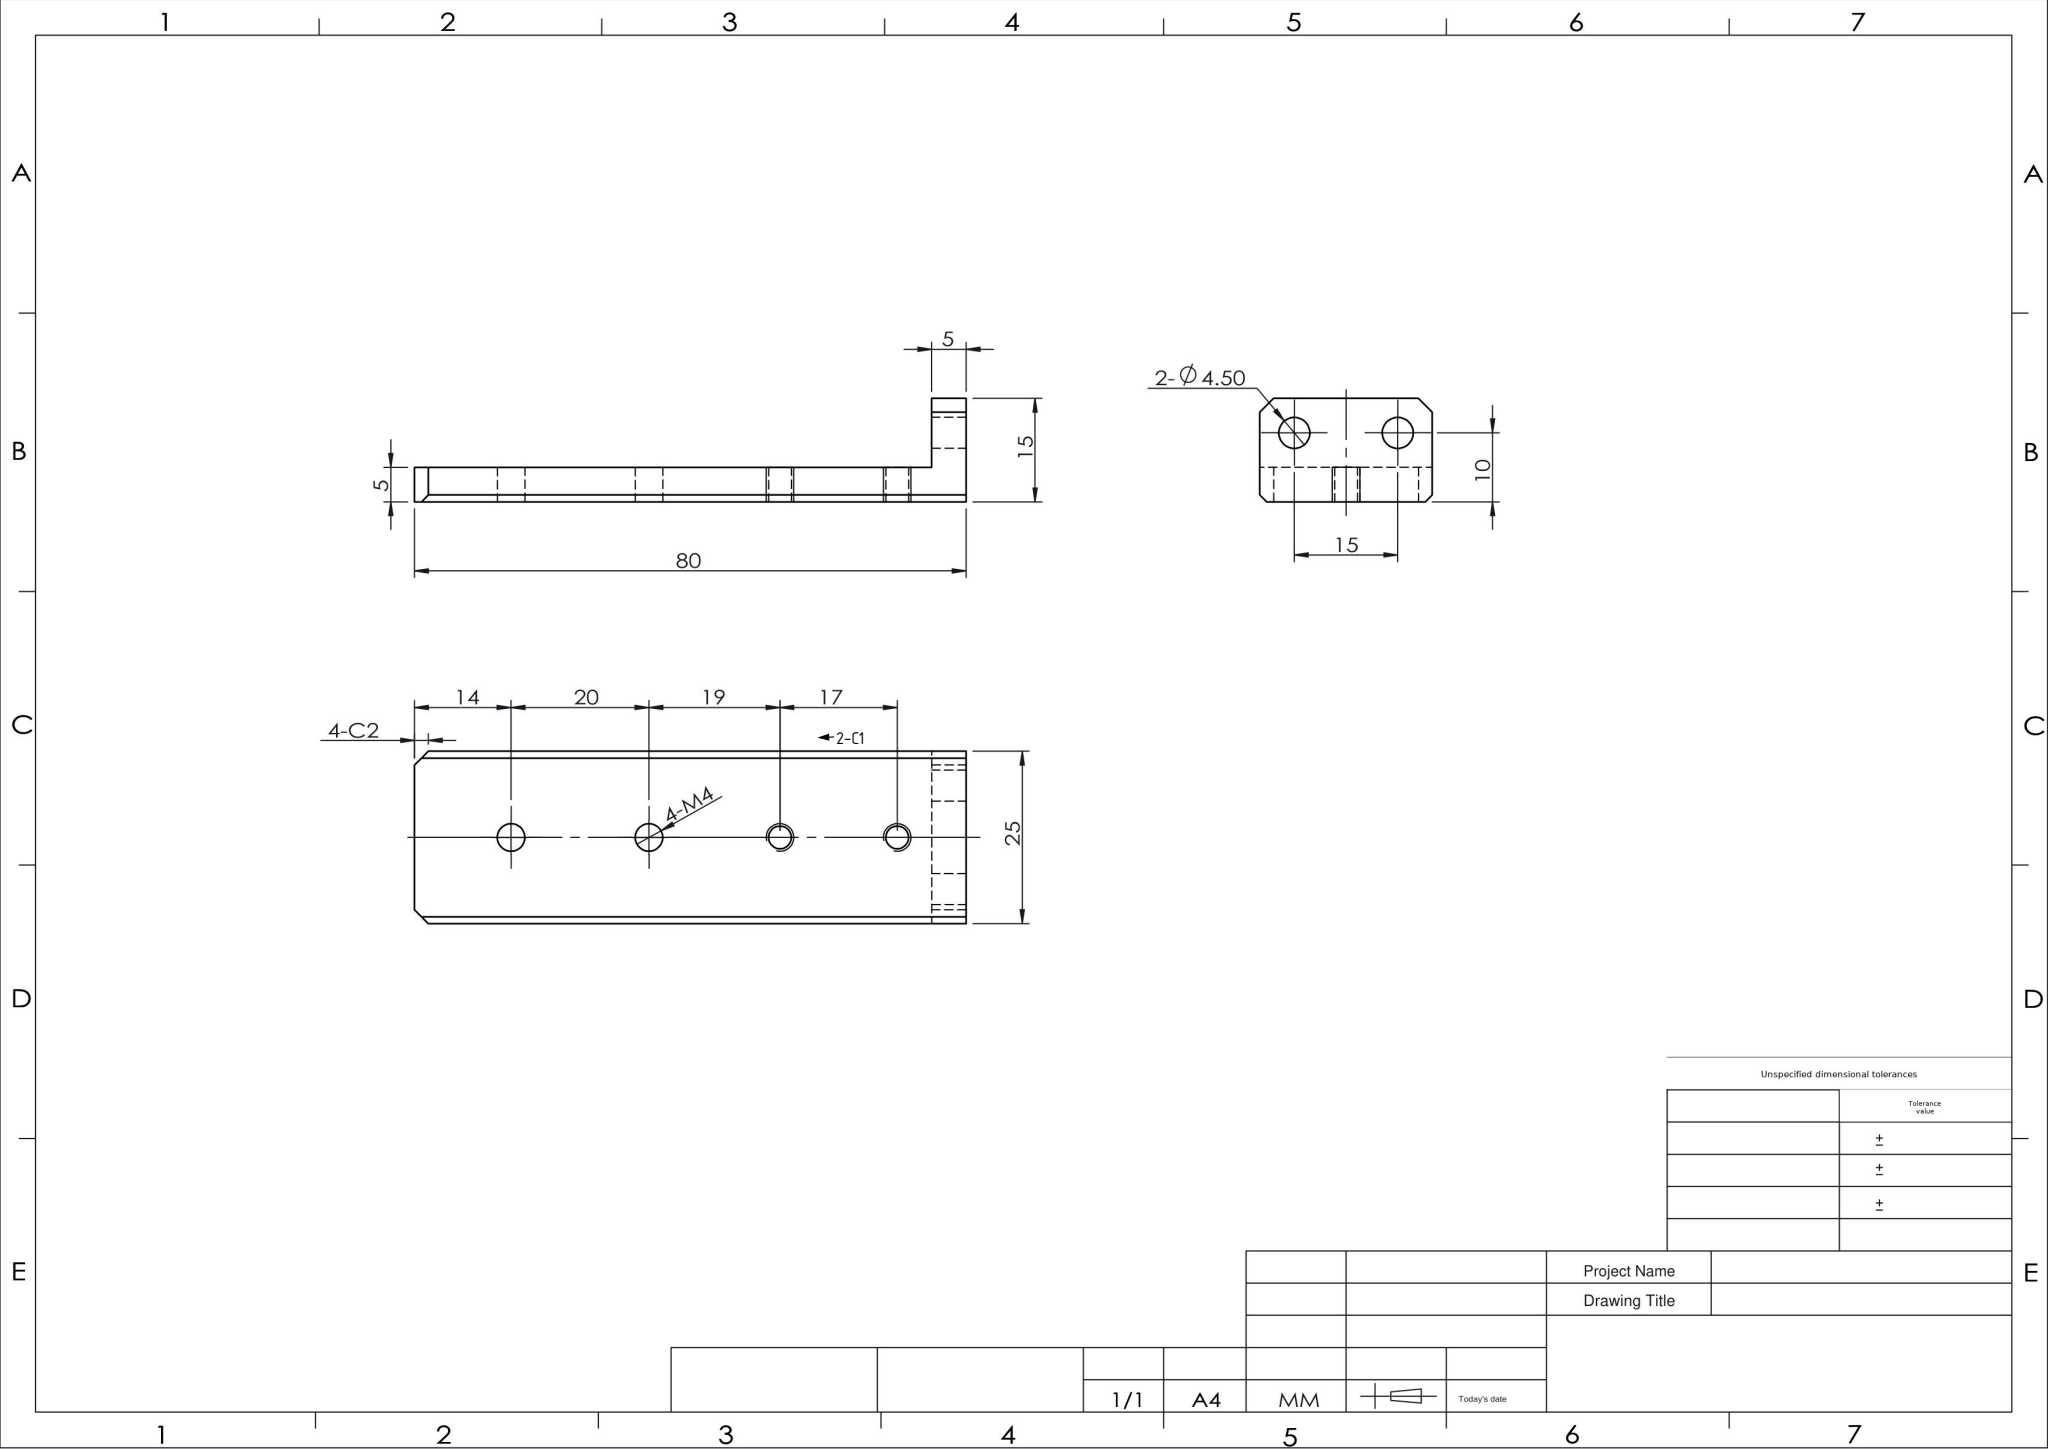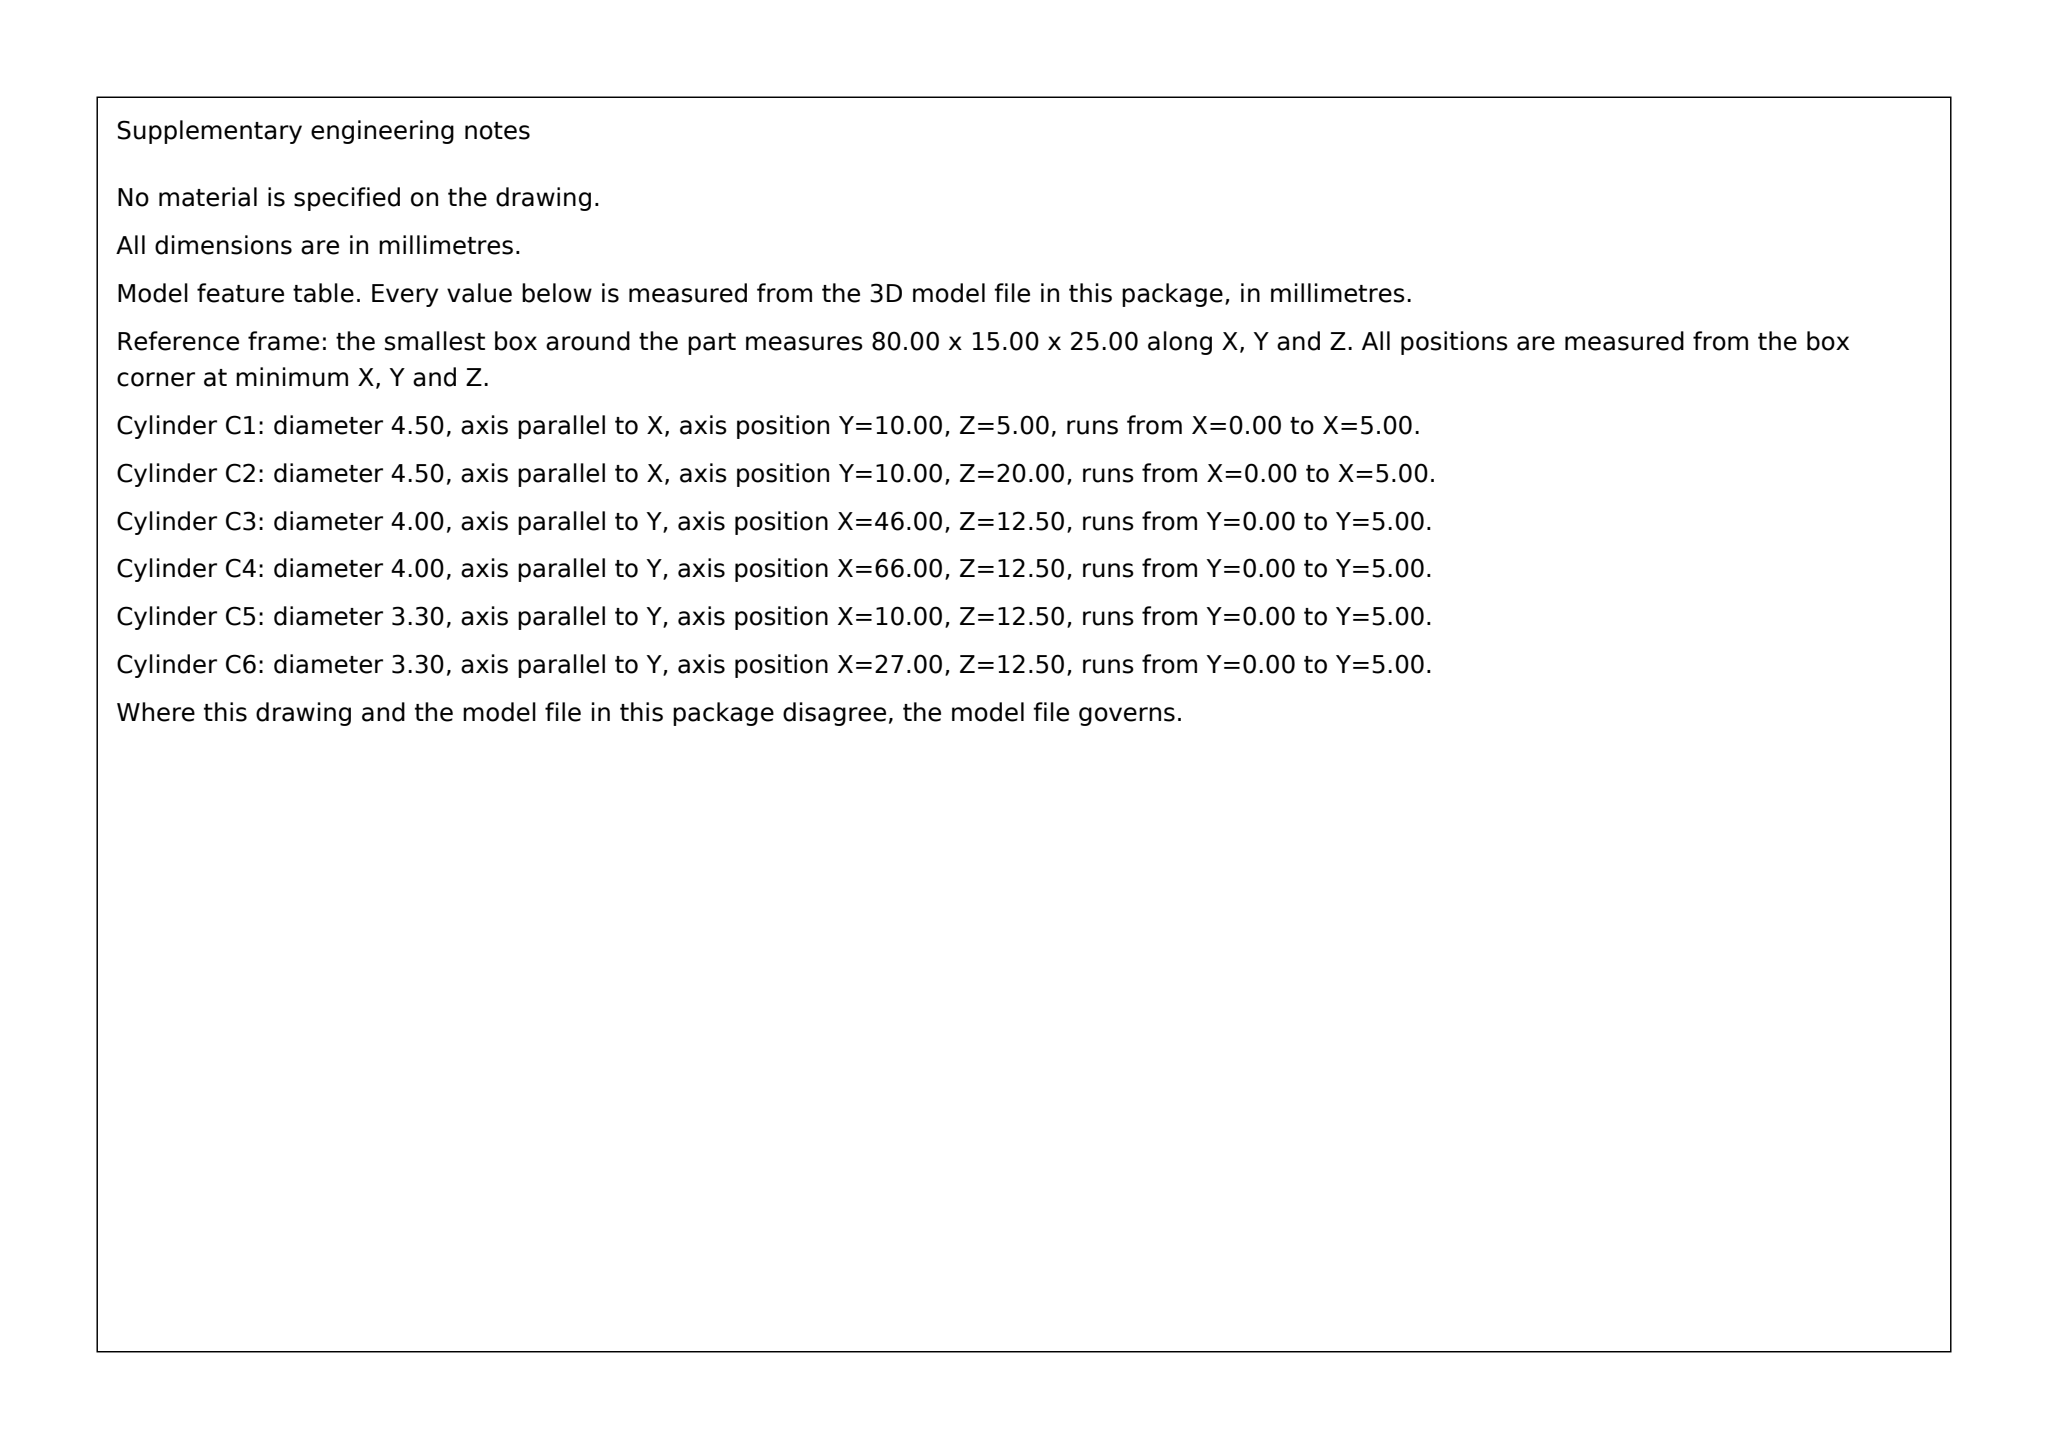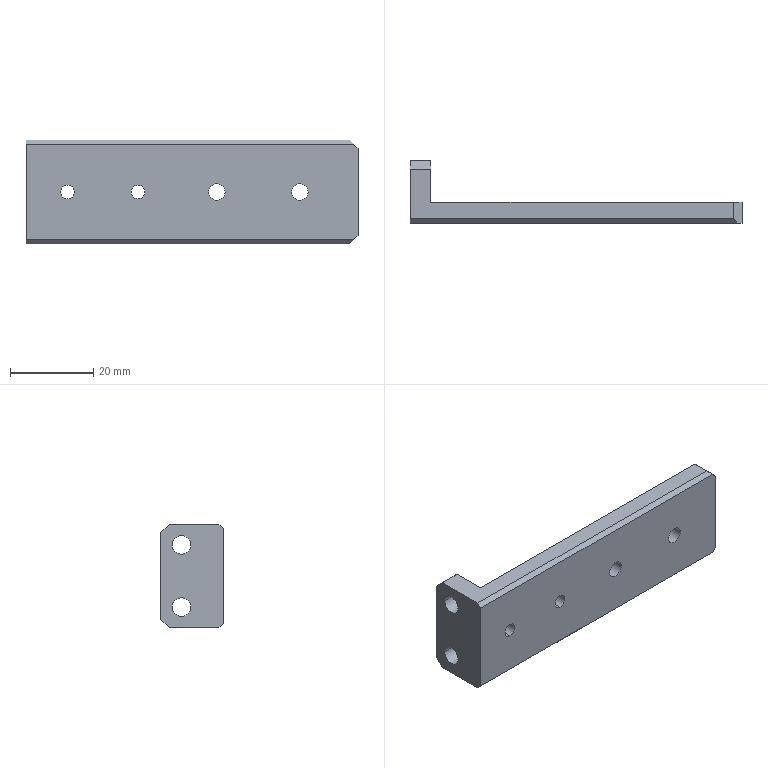Part | SolidWorks | mm | 1 solid | 26 faces | box 80 x 15 x 25 mm | volume 10761 mm3 | plane 14 | cylinder 12 | commonest cylinder face diameters 3.3 x4 4 x4 4.5 x4
Drawing notes:
2-C1 ON LONG BOTTOM EDGES OF 80 ARM (FRONT FACE, FULL 79 LG) | from the solid: Inclined planes 45/45 at bbox_from [0,0,0] and [0,0,24], size [79,1,1] -> 1x1 chamfers along x on y=0 face at z=0 and z=25
build123d program:
from build123d import *

# Parameters (mm, degrees)
BOSS_EXTRUDE1_DEPTH   = 25
SKETCH2_R             = 2.25
CUT_EXTRUDE1_DEPTH    = 81.467
CHAMFER1_SIZE         = 2
SKETCH3_R             = 2
CUT_EXTRUDE2_DEPTH    = 10
M4_TAPPED_HOLE1_D     = 3.3
M4_TAPPED_HOLE1_DEPTH = 10.1
M4_TAPPED_HOLE1_TIP   = 0.9914
CHAMFER2_SIZE         = 1


with BuildPart() as part:
    # Sketch1 → Boss-Extrude1 (new body)
    with BuildSketch(Plane.XY):
        Polygon((0, 15), (5, 15), (5, 5), (80, 5), (80, 0), (0, 0), align=None)
    extrude(amount=BOSS_EXTRUDE1_DEPTH)

    # Sketch2 → Cut-Extrude1 (cut, through all)
    with BuildSketch(Plane(origin=(5, 0, 0), x_dir=(0, 0, -1), z_dir=(1, 0, 0))):
        with Locations(Location((-20, 10, 0), (0, 0, 90))):
            Circle(SKETCH2_R)
        with Locations(Location((-5, 10, 0), (0, 0, 90))):
            Circle(SKETCH2_R)
    extrude(amount=-CUT_EXTRUDE1_DEPTH, mode=Mode.SUBTRACT)

    # Chamfer1
    chamfer1_edges = [part.edges().sort_by_distance(p)[0] for p in [
        (80, 2.5, 25),
        (2.5, 15, 25),
        (2.5, 15, 0),
        (80, 2.5, 0),
    ]]
    chamfer(chamfer1_edges, length=CHAMFER1_SIZE)

    # Sketch3 → Cut-Extrude2 (cut)
    with BuildSketch(Plane(origin=(0, 5, 0), x_dir=(1, 0, 0), z_dir=(0, 1, 0))):
        with Locations(Location((46, -12.5, 0), (0, 0, 180))):
            Circle(SKETCH3_R)
        with Locations(Location((66, -12.5, 0), (0, 0, 180))):
            Circle(SKETCH3_R)
    extrude(amount=-CUT_EXTRUDE2_DEPTH, mode=Mode.SUBTRACT)

    # M4 Tapped Hole1
    with Locations(Plane(origin=(0, 0, 0), x_dir=(-1, 0, 0), z_dir=(0, -1, 0))):
        with Locations((-10, -12.5), (-27, -12.5)):
            Hole(M4_TAPPED_HOLE1_D / 2, depth=M4_TAPPED_HOLE1_DEPTH)
            with Locations((0, 0, -(M4_TAPPED_HOLE1_DEPTH + M4_TAPPED_HOLE1_TIP / 2))):  # 118° drill point
                Cone(0, M4_TAPPED_HOLE1_D / 2, M4_TAPPED_HOLE1_TIP, mode=Mode.SUBTRACT)

    # Chamfer2
    chamfer2_edges = [part.edges().sort_by_distance(p)[0] for p in [
        (39, 0, 25),
        (39, 0, 0),
    ]]
    chamfer(chamfer2_edges, length=CHAMFER2_SIZE)


solid = part.part
STEP:
#1=CARTESIAN_POINT('',(10.,5.,14.15));
#2=VERTEX_POINT('',#1);
#3=CARTESIAN_POINT('',(10.,5.,10.85));
#4=VERTEX_POINT('',#3);
#5=CARTESIAN_POINT('',(10.,5.,12.5));
#6=DIRECTION('',(0.,-1.,0.));
#7=DIRECTION('',(0.,0.,-1.));
#8=AXIS2_PLACEMENT_3D('',#5,#6,#7);
#9=CIRCLE('',#8,1.65);
#10=EDGE_CURVE('',#2,#4,#9,.T.);
#11=ORIENTED_EDGE('',*,*,#10,.F.);
#12=CARTESIAN_POINT('',(10.,-0.,14.15));
#13=VERTEX_POINT('',#12);
#14=CARTESIAN_POINT('',(10.,0.,14.15));
#15=DIRECTION('',(0.,-1.,0.));
#16=VECTOR('',#15,1000.);
#17=LINE('',#14,#16);
#18=EDGE_CURVE('',#2,#13,#17,.T.);
#19=ORIENTED_EDGE('',*,*,#18,.T.);
#20=CARTESIAN_POINT('',(10.,-0.,10.85));
#21=VERTEX_POINT('',#20);
#22=CARTESIAN_POINT('',(10.,-0.,12.5));
#23=DIRECTION('',(0.,-1.,0.));
#24=DIRECTION('',(0.,0.,-1.));
#25=AXIS2_PLACEMENT_3D('',#22,#23,#24);
#26=CIRCLE('',#25,1.65);
#27=EDGE_CURVE('',#13,#21,#26,.T.);
#28=ORIENTED_EDGE('',*,*,#27,.T.);
#29=CARTESIAN_POINT('',(10.,0.,10.85));
#30=DIRECTION('',(0.,-1.,0.));
#31=VECTOR('',#30,1000.);
#32=LINE('',#29,#31);
#33=EDGE_CURVE('',#4,#21,#32,.T.);
#34=ORIENTED_EDGE('',*,*,#33,.F.);
#35=EDGE_LOOP('',(#11,#19,#28,#34));
#36=FACE_OUTER_BOUND('',#35,.T.);
#37=CARTESIAN_POINT('',(10.,0.,12.5));
#38=DIRECTION('',(0.,-1.,0.));
#39=DIRECTION('',(0.,0.,-1.));
#40=AXIS2_PLACEMENT_3D('',#37,#38,#39);
#41=CYLINDRICAL_SURFACE('',#40,1.65);
#42=ADVANCED_FACE('',(#36),#41,.F.);
#43=CARTESIAN_POINT('',(27.,5.,14.15));
#44=VERTEX_POINT('',#43);
#45=CARTESIAN_POINT('',(27.,5.,10.85));
#46=VERTEX_POINT('',#45);
#47=CARTESIAN_POINT('',(27.,5.,12.5));
#48=DIRECTION('',(0.,-1.,0.));
#49=DIRECTION('',(0.,0.,-1.));
#50=AXIS2_PLACEMENT_3D('',#47,#48,#49);
#51=CIRCLE('',#50,1.65);
#52=EDGE_CURVE('',#44,#46,#51,.T.);
#53=ORIENTED_EDGE('',*,*,#52,.F.);
#54=CARTESIAN_POINT('',(27.,-0.,14.15));
#55=VERTEX_POINT('',#54);
#56=CARTESIAN_POINT('',(27.,0.,14.15));
#57=DIRECTION('',(0.,-1.,0.));
#58=VECTOR('',#57,1000.);
#59=LINE('',#56,#58);
#60=EDGE_CURVE('',#44,#55,#59,.T.);
#61=ORIENTED_EDGE('',*,*,#60,.T.);
#62=CARTESIAN_POINT('',(27.,-0.,10.85));
#63=VERTEX_POINT('',#62);
#64=CARTESIAN_POINT('',(27.,-0.,12.5));
#65=DIRECTION('',(0.,-1.,0.));
#66=DIRECTION('',(0.,0.,-1.));
#67=AXIS2_PLACEMENT_3D('',#64,#65,#66);
#68=CIRCLE('',#67,1.65);
#69=EDGE_CURVE('',#55,#63,#68,.T.);
#70=ORIENTED_EDGE('',*,*,#69,.T.);
#71=CARTESIAN_POINT('',(27.,0.,10.85));
#72=DIRECTION('',(0.,-1.,0.));
#73=VECTOR('',#72,1000.);
#74=LINE('',#71,#73);
#75=EDGE_CURVE('',#46,#63,#74,.T.);
#76=ORIENTED_EDGE('',*,*,#75,.F.);
#77=EDGE_LOOP('',(#53,#61,#70,#76));
#78=FACE_OUTER_BOUND('',#77,.T.);
#79=CARTESIAN_POINT('',(27.,0.,12.5));
#80=DIRECTION('',(0.,-1.,0.));
#81=DIRECTION('',(0.,0.,-1.));
#82=AXIS2_PLACEMENT_3D('',#79,#80,#81);
#83=CYLINDRICAL_SURFACE('',#82,1.65);
#84=ADVANCED_FACE('',(#78),#83,.F.);
#85=CARTESIAN_POINT('',(68.,0.,12.5));
#86=VERTEX_POINT('',#85);
#87=CARTESIAN_POINT('',(64.,0.,12.5));
#88=VERTEX_POINT('',#87);
#89=CARTESIAN_POINT('',(66.,0.,12.5));
#90=DIRECTION('',(0.,1.,0.));
#91=DIRECTION('',(0.,0.,1.));
#92=AXIS2_PLACEMENT_3D('',#89,#90,#91);
#93=CIRCLE('',#92,2.);
#94=EDGE_CURVE('',#86,#88,#93,.T.);
#95=ORIENTED_EDGE('',*,*,#94,.F.);
#96=CARTESIAN_POINT('',(68.,5.,12.5));
#97=VERTEX_POINT('',#96);
#98=CARTESIAN_POINT('',(68.,-5.,12.5));
#99=DIRECTION('',(-0.,1.,0.));
#100=VECTOR('',#99,1000.);
#101=LINE('',#98,#100);
#102=EDGE_CURVE('',#86,#97,#101,.T.);
#103=ORIENTED_EDGE('',*,*,#102,.T.);
#104=CARTESIAN_POINT('',(64.,5.,12.5));
#105=VERTEX_POINT('',#104);
#106=CARTESIAN_POINT('',(66.,5.,12.5));
#107=DIRECTION('',(-0.,1.,0.));
#108=DIRECTION('',(-1.,0.,0.));
#109=AXIS2_PLACEMENT_3D('',#106,#107,#108);
#110=CIRCLE('',#109,2.);
#111=EDGE_CURVE('',#97,#105,#110,.T.);
#112=ORIENTED_EDGE('',*,*,#111,.T.);
#113=CARTESIAN_POINT('',(64.,-5.,12.5));
#114=DIRECTION('',(-0.,1.,0.));
#115=VECTOR('',#114,1000.);
#116=LINE('',#113,#115);
#117=EDGE_CURVE('',#88,#105,#116,.T.);
#118=ORIENTED_EDGE('',*,*,#117,.F.);
#119=EDGE_LOOP('',(#95,#103,#112,#118));
#120=FACE_OUTER_BOUND('',#119,.T.);
#121=CARTESIAN_POINT('',(66.,-5.,12.5));
#122=DIRECTION('',(-0.,1.,0.));
#123=DIRECTION('',(-1.,0.,0.));
#124=AXIS2_PLACEMENT_3D('',#121,#122,#123);
#125=CYLINDRICAL_SURFACE('',#124,2.);
#126=ADVANCED_FACE('',(#120),#125,.F.);
#127=CARTESIAN_POINT('',(48.,0.,12.5));
#128=VERTEX_POINT('',#127);
#129=CARTESIAN_POINT('',(44.,0.,12.5));
#130=VERTEX_POINT('',#129);
#131=CARTESIAN_POINT('',(46.,0.,12.5));
#132=DIRECTION('',(0.,1.,0.));
#133=DIRECTION('',(0.,0.,1.));
#134=AXIS2_PLACEMENT_3D('',#131,#132,#133);
#135=CIRCLE('',#134,2.);
#136=EDGE_CURVE('',#128,#130,#135,.T.);
#137=ORIENTED_EDGE('',*,*,#136,.F.);
#138=CARTESIAN_POINT('',(48.,5.,12.5));
#139=VERTEX_POINT('',#138);
#140=CARTESIAN_POINT('',(48.,-5.,12.5));
#141=DIRECTION('',(-0.,1.,0.));
#142=VECTOR('',#141,1000.);
#143=LINE('',#140,#142);
#144=EDGE_CURVE('',#128,#139,#143,.T.);
#145=ORIENTED_EDGE('',*,*,#144,.T.);
#146=CARTESIAN_POINT('',(44.,5.,12.5));
#147=VERTEX_POINT('',#146);
#148=CARTESIAN_POINT('',(46.,5.,12.5));
#149=DIRECTION('',(-0.,1.,0.));
#150=DIRECTION('',(-1.,0.,0.));
#151=AXIS2_PLACEMENT_3D('',#148,#149,#150);
#152=CIRCLE('',#151,2.);
#153=EDGE_CURVE('',#139,#147,#152,.T.);
#154=ORIENTED_EDGE('',*,*,#153,.T.);
#155=CARTESIAN_POINT('',(44.,-5.,12.5));
#156=DIRECTION('',(-0.,1.,0.));
#157=VECTOR('',#156,1000.);
#158=LINE('',#155,#157);
#159=EDGE_CURVE('',#130,#147,#158,.T.);
#160=ORIENTED_EDGE('',*,*,#159,.F.);
#161=EDGE_LOOP('',(#137,#145,#154,#160));
#162=FACE_OUTER_BOUND('',#161,.T.);
#163=CARTESIAN_POINT('',(46.,-5.,12.5));
#164=DIRECTION('',(-0.,1.,0.));
#165=DIRECTION('',(-1.,0.,0.));
#166=AXIS2_PLACEMENT_3D('',#163,#164,#165);
#167=CYLINDRICAL_SURFACE('',#166,2.);
#168=ADVANCED_FACE('',(#162),#167,.F.);
#169=CARTESIAN_POINT('',(-0.,7.75,5.));
#170=VERTEX_POINT('',#169);
#171=CARTESIAN_POINT('',(-0.,12.25,5.));
#172=VERTEX_POINT('',#171);
#173=CARTESIAN_POINT('',(-0.,10.,5.));
#174=DIRECTION('',(1.,0.,0.));
#175=DIRECTION('',(-0.,1.,0.));
#176=AXIS2_PLACEMENT_3D('',#173,#174,#175);
#177=CIRCLE('',#176,2.25);
#178=EDGE_CURVE('',#170,#172,#177,.T.);
#179=ORIENTED_EDGE('',*,*,#178,.F.);
#180=CARTESIAN_POINT('',(5.,7.75,5.));
#181=VERTEX_POINT('',#180);
#182=CARTESIAN_POINT('',(-0.,7.75,5.));
#183=DIRECTION('',(1.,0.,0.));
#184=VECTOR('',#183,1000.);
#185=LINE('',#182,#184);
#186=EDGE_CURVE('',#170,#181,#185,.T.);
#187=ORIENTED_EDGE('',*,*,#186,.T.);
#188=CARTESIAN_POINT('',(5.,12.25,5.));
#189=VERTEX_POINT('',#188);
#190=CARTESIAN_POINT('',(5.,10.,5.));
#191=DIRECTION('',(1.,0.,0.));
#192=DIRECTION('',(-0.,1.,0.));
#193=AXIS2_PLACEMENT_3D('',#190,#191,#192);
#194=CIRCLE('',#193,2.25);
#195=EDGE_CURVE('',#181,#189,#194,.T.);
#196=ORIENTED_EDGE('',*,*,#195,.T.);
#197=CARTESIAN_POINT('',(-0.,12.25,5.));
#198=DIRECTION('',(1.,0.,0.));
#199=VECTOR('',#198,1000.);
#200=LINE('',#197,#199);
#201=EDGE_CURVE('',#172,#189,#200,.T.);
#202=ORIENTED_EDGE('',*,*,#201,.F.);
#203=EDGE_LOOP('',(#179,#187,#196,#202));
#204=FACE_OUTER_BOUND('',#203,.T.);
#205=CARTESIAN_POINT('',(-0.,10.,5.));
#206=DIRECTION('',(1.,0.,0.));
#207=DIRECTION('',(-0.,1.,0.));
#208=AXIS2_PLACEMENT_3D('',#205,#206,#207);
#209=CYLINDRICAL_SURFACE('',#208,2.25);
#210=ADVANCED_FACE('',(#204),#209,.F.);
#211=CARTESIAN_POINT('',(-0.,7.75,20.));
#212=VERTEX_POINT('',#211);
#213=CARTESIAN_POINT('',(-0.,12.25,20.));
#214=VERTEX_POINT('',#213);
#215=CARTESIAN_POINT('',(-0.,10.,20.));
#216=DIRECTION('',(1.,0.,0.));
#217=DIRECTION('',(-0.,1.,0.));
#218=AXIS2_PLACEMENT_3D('',#215,#216,#217);
#219=CIRCLE('',#218,2.25);
#220=EDGE_CURVE('',#212,#214,#219,.T.);
#221=ORIENTED_EDGE('',*,*,#220,.F.);
#222=CARTESIAN_POINT('',(5.,7.75,20.));
#223=VERTEX_POINT('',#222);
#224=CARTESIAN_POINT('',(-0.,7.75,20.));
#225=DIRECTION('',(1.,0.,0.));
#226=VECTOR('',#225,1000.);
#227=LINE('',#224,#226);
#228=EDGE_CURVE('',#212,#223,#227,.T.);
#229=ORIENTED_EDGE('',*,*,#228,.T.);
#230=CARTESIAN_POINT('',(5.,12.25,20.));
#231=VERTEX_POINT('',#230);
#232=CARTESIAN_POINT('',(5.,10.,20.));
#233=DIRECTION('',(1.,0.,0.));
#234=DIRECTION('',(-0.,1.,0.));
#235=AXIS2_PLACEMENT_3D('',#232,#233,#234);
#236=CIRCLE('',#235,2.25);
#237=EDGE_CURVE('',#223,#231,#236,.T.);
#238=ORIENTED_EDGE('',*,*,#237,.T.);
#239=CARTESIAN_POINT('',(-0.,12.25,20.));
#240=DIRECTION('',(1.,0.,0.));
#241=VECTOR('',#240,1000.);
#242=LINE('',#239,#241);
#243=EDGE_CURVE('',#214,#231,#242,.T.);
#244=ORIENTED_EDGE('',*,*,#243,.F.);
#245=EDGE_LOOP('',(#221,#229,#238,#244));
#246=FACE_OUTER_BOUND('',#245,.T.);
#247=CARTESIAN_POINT('',(-0.,10.,20.));
#248=DIRECTION('',(1.,0.,0.));
#249=DIRECTION('',(-0.,1.,0.));
#250=AXIS2_PLACEMENT_3D('',#247,#248,#249);
#251=CYLINDRICAL_SURFACE('',#250,2.25);
#252=ADVANCED_FACE('',(#246),#251,.F.);
#253=CARTESIAN_POINT('',(-0.,10.,5.));
#254=DIRECTION('',(1.,0.,0.));
#255=DIRECTION('',(-0.,1.,0.));
#256=AXIS2_PLACEMENT_3D('',#253,#254,#255);
#257=CIRCLE('',#256,2.25);
#258=EDGE_CURVE('',#172,#170,#257,.T.);
#259=ORIENTED_EDGE('',*,*,#258,.T.);
#260=ORIENTED_EDGE('',*,*,#178,.T.);
#261=EDGE_LOOP('',(#259,#260));
#262=FACE_BOUND('',#261,.T.);
#263=CARTESIAN_POINT('',(-0.,10.,20.));
#264=DIRECTION('',(1.,0.,0.));
#265=DIRECTION('',(-0.,1.,0.));
#266=AXIS2_PLACEMENT_3D('',#263,#264,#265);
#267=CIRCLE('',#266,2.25);
#268=EDGE_CURVE('',#214,#212,#267,.T.);
#269=ORIENTED_EDGE('',*,*,#268,.T.);
#270=ORIENTED_EDGE('',*,*,#220,.T.);
#271=EDGE_LOOP('',(#269,#270));
#272=FACE_BOUND('',#271,.T.);
#273=CARTESIAN_POINT('',(-0.,-0.,24.));
#274=VERTEX_POINT('',#273);
#275=CARTESIAN_POINT('',(-0.,-0.,1.));
#276=VERTEX_POINT('',#275);
#277=CARTESIAN_POINT('',(0.,0.,25.));
#278=DIRECTION('',(0.,0.,-1.));
#279=VECTOR('',#278,1000.);
#280=LINE('',#277,#279);
#281=EDGE_CURVE('',#274,#276,#280,.T.);
#282=ORIENTED_EDGE('',*,*,#281,.F.);
#283=CARTESIAN_POINT('',(0.,1.,25.));
#284=VERTEX_POINT('',#283);
#285=CARTESIAN_POINT('',(0.,1.,25.));
#286=DIRECTION('',(0.,0.7071,0.7071));
#287=VECTOR('',#286,1000.);
#288=LINE('',#285,#287);
#289=EDGE_CURVE('',#274,#284,#288,.T.);
#290=ORIENTED_EDGE('',*,*,#289,.T.);
#291=CARTESIAN_POINT('',(0.,13.,25.));
#292=VERTEX_POINT('',#291);
#293=CARTESIAN_POINT('',(0.,15.,25.));
#294=DIRECTION('',(-0.,-1.,0.));
#295=VECTOR('',#294,1000.);
#296=LINE('',#293,#295);
#297=EDGE_CURVE('',#292,#284,#296,.T.);
#298=ORIENTED_EDGE('',*,*,#297,.F.);
#299=CARTESIAN_POINT('',(0.,15.,23.));
#300=VERTEX_POINT('',#299);
#301=CARTESIAN_POINT('',(0.,13.,25.));
#302=DIRECTION('',(0.,0.7071,-0.7071));
#303=VECTOR('',#302,1000.);
#304=LINE('',#301,#303);
#305=EDGE_CURVE('',#292,#300,#304,.T.);
#306=ORIENTED_EDGE('',*,*,#305,.T.);
#307=CARTESIAN_POINT('',(0.,15.,2.));
#308=VERTEX_POINT('',#307);
#309=CARTESIAN_POINT('',(0.,15.,25.));
#310=DIRECTION('',(0.,0.,-1.));
#311=VECTOR('',#310,1000.);
#312=LINE('',#309,#311);
#313=EDGE_CURVE('',#300,#308,#312,.T.);
#314=ORIENTED_EDGE('',*,*,#313,.T.);
#315=CARTESIAN_POINT('',(0.,13.,0.));
#316=VERTEX_POINT('',#315);
#317=CARTESIAN_POINT('',(0.,15.,2.));
#318=DIRECTION('',(-0.,-0.7071,-0.7071));
#319=VECTOR('',#318,1000.);
#320=LINE('',#317,#319);
#321=EDGE_CURVE('',#308,#316,#320,.T.);
#322=ORIENTED_EDGE('',*,*,#321,.T.);
#323=CARTESIAN_POINT('',(0.,1.,-0.));
#324=VERTEX_POINT('',#323);
#325=CARTESIAN_POINT('',(0.,15.,0.));
#326=DIRECTION('',(-0.,-1.,0.));
#327=VECTOR('',#326,1000.);
#328=LINE('',#325,#327);
#329=EDGE_CURVE('',#316,#324,#328,.T.);
#330=ORIENTED_EDGE('',*,*,#329,.T.);
#331=CARTESIAN_POINT('',(-0.,0.,1.));
#332=DIRECTION('',(-0.,-0.7071,0.7071));
#333=VECTOR('',#332,1000.);
#334=LINE('',#331,#333);
#335=EDGE_CURVE('',#324,#276,#334,.T.);
#336=ORIENTED_EDGE('',*,*,#335,.T.);
#337=EDGE_LOOP('',(#282,#290,#298,#306,#314,#322,#330,#336));
#338=FACE_OUTER_BOUND('',#337,.T.);
#339=CARTESIAN_POINT('',(0.,15.,25.));
#340=DIRECTION('',(1.,-0.,0.));
#341=DIRECTION('',(0.,1.,0.));
#342=AXIS2_PLACEMENT_3D('',#339,#340,#341);
#343=PLANE('',#342);
#344=ADVANCED_FACE('',(#262,#272,#338),#343,.F.);
#345=CARTESIAN_POINT('',(10.,-0.,12.5));
#346=DIRECTION('',(0.,-1.,0.));
#347=DIRECTION('',(0.,0.,-1.));
#348=AXIS2_PLACEMENT_3D('',#345,#346,#347);
#349=CIRCLE('',#348,1.65);
#350=EDGE_CURVE('',#21,#13,#349,.T.);
#351=ORIENTED_EDGE('',*,*,#350,.F.);
#352=ORIENTED_EDGE('',*,*,#27,.F.);
#353=EDGE_LOOP('',(#351,#352));
#354=FACE_BOUND('',#353,.T.);
#355=CARTESIAN_POINT('',(27.,-0.,12.5));
#356=DIRECTION('',(0.,-1.,0.));
#357=DIRECTION('',(0.,0.,-1.));
#358=AXIS2_PLACEMENT_3D('',#355,#356,#357);
#359=CIRCLE('',#358,1.65);
#360=EDGE_CURVE('',#63,#55,#359,.T.);
#361=ORIENTED_EDGE('',*,*,#360,.F.);
#362=ORIENTED_EDGE('',*,*,#69,.F.);
#363=EDGE_LOOP('',(#361,#362));
#364=FACE_BOUND('',#363,.T.);
#365=CARTESIAN_POINT('',(66.,0.,12.5));
#366=DIRECTION('',(0.,1.,0.));
#367=DIRECTION('',(0.,0.,1.));
#368=AXIS2_PLACEMENT_3D('',#365,#366,#367);
#369=CIRCLE('',#368,2.);
#370=EDGE_CURVE('',#88,#86,#369,.T.);
#371=ORIENTED_EDGE('',*,*,#370,.T.);
#372=ORIENTED_EDGE('',*,*,#94,.T.);
#373=EDGE_LOOP('',(#371,#372));
#374=FACE_BOUND('',#373,.T.);
#375=CARTESIAN_POINT('',(46.,0.,12.5));
#376=DIRECTION('',(0.,1.,0.));
#377=DIRECTION('',(0.,0.,1.));
#378=AXIS2_PLACEMENT_3D('',#375,#376,#377);
#379=CIRCLE('',#378,2.);
#380=EDGE_CURVE('',#130,#128,#379,.T.);
#381=ORIENTED_EDGE('',*,*,#380,.T.);
#382=ORIENTED_EDGE('',*,*,#136,.T.);
#383=EDGE_LOOP('',(#381,#382));
#384=FACE_BOUND('',#383,.T.);
#385=CARTESIAN_POINT('',(80.,0.,23.));
#386=VERTEX_POINT('',#385);
#387=CARTESIAN_POINT('',(79.,0.,24.));
#388=VERTEX_POINT('',#387);
#389=CARTESIAN_POINT('',(78.,0.,25.));
#390=DIRECTION('',(-0.7071,0.,0.7071));
#391=VECTOR('',#390,1000.);
#392=LINE('',#389,#391);
#393=EDGE_CURVE('',#386,#388,#392,.T.);
#394=ORIENTED_EDGE('',*,*,#393,.T.);
#395=CARTESIAN_POINT('',(0.,0.,24.));
#396=DIRECTION('',(-1.,0.,0.));
#397=VECTOR('',#396,1000.);
#398=LINE('',#395,#397);
#399=EDGE_CURVE('',#388,#274,#398,.T.);
#400=ORIENTED_EDGE('',*,*,#399,.T.);
#401=ORIENTED_EDGE('',*,*,#281,.T.);
#402=CARTESIAN_POINT('',(79.,0.,1.));
#403=VERTEX_POINT('',#402);
#404=CARTESIAN_POINT('',(0.,0.,1.));
#405=DIRECTION('',(1.,0.,0.));
#406=VECTOR('',#405,1000.);
#407=LINE('',#404,#406);
#408=EDGE_CURVE('',#276,#403,#407,.T.);
#409=ORIENTED_EDGE('',*,*,#408,.T.);
#410=CARTESIAN_POINT('',(80.,0.,2.));
#411=VERTEX_POINT('',#410);
#412=CARTESIAN_POINT('',(80.,0.,2.));
#413=DIRECTION('',(0.7071,0.,0.7071));
#414=VECTOR('',#413,1000.);
#415=LINE('',#412,#414);
#416=EDGE_CURVE('',#403,#411,#415,.T.);
#417=ORIENTED_EDGE('',*,*,#416,.T.);
#418=CARTESIAN_POINT('',(80.,0.,25.));
#419=DIRECTION('',(0.,0.,-1.));
#420=VECTOR('',#419,1000.);
#421=LINE('',#418,#420);
#422=EDGE_CURVE('',#386,#411,#421,.T.);
#423=ORIENTED_EDGE('',*,*,#422,.F.);
#424=EDGE_LOOP('',(#394,#400,#401,#409,#417,#423));
#425=FACE_OUTER_BOUND('',#424,.T.);
#426=CARTESIAN_POINT('',(0.,0.,25.));
#427=DIRECTION('',(0.,1.,0.));
#428=DIRECTION('',(0.,0.,1.));
#429=AXIS2_PLACEMENT_3D('',#426,#427,#428);
#430=PLANE('',#429);
#431=ADVANCED_FACE('',(#354,#364,#374,#384,#425),#430,.F.);
#432=ORIENTED_EDGE('',*,*,#422,.T.);
#433=CARTESIAN_POINT('',(80.,5.,2.));
#434=VERTEX_POINT('',#433);
#435=CARTESIAN_POINT('',(80.,5.,2.));
#436=DIRECTION('',(0.,1.,0.));
#437=VECTOR('',#436,1000.);
#438=LINE('',#435,#437);
#439=EDGE_CURVE('',#411,#434,#438,.T.);
#440=ORIENTED_EDGE('',*,*,#439,.T.);
#441=CARTESIAN_POINT('',(80.,5.,23.));
#442=VERTEX_POINT('',#441);
#443=CARTESIAN_POINT('',(80.,5.,25.));
#444=DIRECTION('',(0.,0.,-1.));
#445=VECTOR('',#444,1000.);
#446=LINE('',#443,#445);
#447=EDGE_CURVE('',#442,#434,#446,.T.);
#448=ORIENTED_EDGE('',*,*,#447,.F.);
#449=CARTESIAN_POINT('',(80.,0.,23.));
#450=DIRECTION('',(0.,-1.,0.));
#451=VECTOR('',#450,1000.);
#452=LINE('',#449,#451);
#453=EDGE_CURVE('',#442,#386,#452,.T.);
#454=ORIENTED_EDGE('',*,*,#453,.T.);
#455=EDGE_LOOP('',(#432,#440,#448,#454));
#456=FACE_OUTER_BOUND('',#455,.T.);
#457=CARTESIAN_POINT('',(80.,5.,25.));
#458=DIRECTION('',(-1.,0.,0.));
#459=DIRECTION('',(0.,0.,1.));
#460=AXIS2_PLACEMENT_3D('',#457,#458,#459);
#461=PLANE('',#460);
#462=ADVANCED_FACE('',(#456),#461,.F.);
#463=CARTESIAN_POINT('',(10.,5.,12.5));
#464=DIRECTION('',(0.,-1.,0.));
#465=DIRECTION('',(0.,0.,-1.));
#466=AXIS2_PLACEMENT_3D('',#463,#464,#465);
#467=CIRCLE('',#466,1.65);
#468=EDGE_CURVE('',#4,#2,#467,.T.);
#469=ORIENTED_EDGE('',*,*,#468,.T.);
#470=ORIENTED_EDGE('',*,*,#10,.T.);
#471=EDGE_LOOP('',(#469,#470));
#472=FACE_BOUND('',#471,.T.);
#473=CARTESIAN_POINT('',(27.,5.,12.5));
#474=DIRECTION('',(0.,-1.,0.));
#475=DIRECTION('',(0.,0.,-1.));
#476=AXIS2_PLACEMENT_3D('',#473,#474,#475);
#477=CIRCLE('',#476,1.65);
#478=EDGE_CURVE('',#46,#44,#477,.T.);
#479=ORIENTED_EDGE('',*,*,#478,.T.);
#480=ORIENTED_EDGE('',*,*,#52,.T.);
#481=EDGE_LOOP('',(#479,#480));
#482=FACE_BOUND('',#481,.T.);
#483=CARTESIAN_POINT('',(66.,5.,12.5));
#484=DIRECTION('',(-0.,1.,0.));
#485=DIRECTION('',(-1.,0.,0.));
#486=AXIS2_PLACEMENT_3D('',#483,#484,#485);
#487=CIRCLE('',#486,2.);
#488=EDGE_CURVE('',#105,#97,#487,.T.);
#489=ORIENTED_EDGE('',*,*,#488,.F.);
#490=ORIENTED_EDGE('',*,*,#111,.F.);
#491=EDGE_LOOP('',(#489,#490));
#492=FACE_BOUND('',#491,.T.);
#493=CARTESIAN_POINT('',(46.,5.,12.5));
#494=DIRECTION('',(-0.,1.,0.));
#495=DIRECTION('',(-1.,0.,0.));
#496=AXIS2_PLACEMENT_3D('',#493,#494,#495);
#497=CIRCLE('',#496,2.);
#498=EDGE_CURVE('',#147,#139,#497,.T.);
#499=ORIENTED_EDGE('',*,*,#498,.F.);
#500=ORIENTED_EDGE('',*,*,#153,.F.);
#501=EDGE_LOOP('',(#499,#500));
#502=FACE_BOUND('',#501,.T.);
#503=ORIENTED_EDGE('',*,*,#447,.T.);
#504=CARTESIAN_POINT('',(78.,5.,0.));
#505=VERTEX_POINT('',#504);
#506=CARTESIAN_POINT('',(80.,5.,2.));
#507=DIRECTION('',(-0.7071,0.,-0.7071));
#508=VECTOR('',#507,1000.);
#509=LINE('',#506,#508);
#510=EDGE_CURVE('',#434,#505,#509,.T.);
#511=ORIENTED_EDGE('',*,*,#510,.T.);
#512=CARTESIAN_POINT('',(5.,5.,0.));
#513=VERTEX_POINT('',#512);
#514=CARTESIAN_POINT('',(5.,5.,0.));
#515=DIRECTION('',(-1.,0.,0.));
#516=VECTOR('',#515,1000.);
#517=LINE('',#514,#516);
#518=EDGE_CURVE('',#505,#513,#517,.T.);
#519=ORIENTED_EDGE('',*,*,#518,.T.);
#520=CARTESIAN_POINT('',(5.,5.,25.));
#521=VERTEX_POINT('',#520);
#522=CARTESIAN_POINT('',(5.,5.,25.));
#523=DIRECTION('',(0.,0.,-1.));
#524=VECTOR('',#523,1000.);
#525=LINE('',#522,#524);
#526=EDGE_CURVE('',#521,#513,#525,.T.);
#527=ORIENTED_EDGE('',*,*,#526,.F.);
#528=CARTESIAN_POINT('',(78.,5.,25.));
#529=VERTEX_POINT('',#528);
#530=CARTESIAN_POINT('',(5.,5.,25.));
#531=DIRECTION('',(-1.,0.,0.));
#532=VECTOR('',#531,1000.);
#533=LINE('',#530,#532);
#534=EDGE_CURVE('',#529,#521,#533,.T.);
#535=ORIENTED_EDGE('',*,*,#534,.F.);
#536=CARTESIAN_POINT('',(78.,5.,25.));
#537=DIRECTION('',(0.7071,0.,-0.7071));
#538=VECTOR('',#537,1000.);
#539=LINE('',#536,#538);
#540=EDGE_CURVE('',#529,#442,#539,.T.);
#541=ORIENTED_EDGE('',*,*,#540,.T.);
#542=EDGE_LOOP('',(#503,#511,#519,#527,#535,#541));
#543=FACE_OUTER_BOUND('',#542,.T.);
#544=CARTESIAN_POINT('',(5.,5.,25.));
#545=DIRECTION('',(0.,-1.,0.));
#546=DIRECTION('',(0.,0.,-1.));
#547=AXIS2_PLACEMENT_3D('',#544,#545,#546);
#548=PLANE('',#547);
#549=ADVANCED_FACE('',(#472,#482,#492,#502,#543),#548,.F.);
#550=CARTESIAN_POINT('',(5.,10.,5.));
#551=DIRECTION('',(1.,0.,0.));
#552=DIRECTION('',(-0.,1.,0.));
#553=AXIS2_PLACEMENT_3D('',#550,#551,#552);
#554=CIRCLE('',#553,2.25);
#555=EDGE_CURVE('',#189,#181,#554,.T.);
#556=ORIENTED_EDGE('',*,*,#555,.F.);
#557=ORIENTED_EDGE('',*,*,#195,.F.);
#558=EDGE_LOOP('',(#556,#557));
#559=FACE_BOUND('',#558,.T.);
#560=CARTESIAN_POINT('',(5.,10.,20.));
#561=DIRECTION('',(1.,0.,0.));
#562=DIRECTION('',(-0.,1.,0.));
#563=AXIS2_PLACEMENT_3D('',#560,#561,#562);
#564=CIRCLE('',#563,2.25);
#565=EDGE_CURVE('',#231,#223,#564,.T.);
#566=ORIENTED_EDGE('',*,*,#565,.F.);
#567=ORIENTED_EDGE('',*,*,#237,.F.);
#568=EDGE_LOOP('',(#566,#567));
#569=FACE_BOUND('',#568,.T.);
#570=CARTESIAN_POINT('',(5.,13.,-0.));
#571=VERTEX_POINT('',#570);
#572=CARTESIAN_POINT('',(5.,15.,0.));
#573=DIRECTION('',(-0.,1.,0.));
#574=VECTOR('',#573,1000.);
#575=LINE('',#572,#574);
#576=EDGE_CURVE('',#513,#571,#575,.T.);
#577=ORIENTED_EDGE('',*,*,#576,.T.);
#578=CARTESIAN_POINT('',(5.,15.,2.));
#579=VERTEX_POINT('',#578);
#580=CARTESIAN_POINT('',(5.,15.,2.));
#581=DIRECTION('',(-0.,0.7071,0.7071));
#582=VECTOR('',#581,1000.);
#583=LINE('',#580,#582);
#584=EDGE_CURVE('',#571,#579,#583,.T.);
#585=ORIENTED_EDGE('',*,*,#584,.T.);
#586=CARTESIAN_POINT('',(5.,15.,23.));
#587=VERTEX_POINT('',#586);
#588=CARTESIAN_POINT('',(5.,15.,25.));
#589=DIRECTION('',(0.,0.,-1.));
#590=VECTOR('',#589,1000.);
#591=LINE('',#588,#590);
#592=EDGE_CURVE('',#587,#579,#591,.T.);
#593=ORIENTED_EDGE('',*,*,#592,.F.);
#594=CARTESIAN_POINT('',(5.,13.,25.));
#595=VERTEX_POINT('',#594);
#596=CARTESIAN_POINT('',(5.,13.,25.));
#597=DIRECTION('',(0.,-0.7071,0.7071));
#598=VECTOR('',#597,1000.);
#599=LINE('',#596,#598);
#600=EDGE_CURVE('',#587,#595,#599,.T.);
#601=ORIENTED_EDGE('',*,*,#600,.T.);
#602=CARTESIAN_POINT('',(5.,15.,25.));
#603=DIRECTION('',(-0.,1.,0.));
#604=VECTOR('',#603,1000.);
#605=LINE('',#602,#604);
#606=EDGE_CURVE('',#521,#595,#605,.T.);
#607=ORIENTED_EDGE('',*,*,#606,.F.);
#608=ORIENTED_EDGE('',*,*,#526,.T.);
#609=EDGE_LOOP('',(#577,#585,#593,#601,#607,#608));
#610=FACE_OUTER_BOUND('',#609,.T.);
#611=CARTESIAN_POINT('',(5.,15.,25.));
#612=DIRECTION('',(-1.,-0.,0.));
#613=DIRECTION('',(0.,-1.,0.));
#614=AXIS2_PLACEMENT_3D('',#611,#612,#613);
#615=PLANE('',#614);
#616=ADVANCED_FACE('',(#559,#569,#610),#615,.F.);
#617=ORIENTED_EDGE('',*,*,#592,.T.);
#618=CARTESIAN_POINT('',(0.,15.,2.));
#619=DIRECTION('',(-1.,0.,0.));
#620=VECTOR('',#619,1000.);
#621=LINE('',#618,#620);
#622=EDGE_CURVE('',#579,#308,#621,.T.);
#623=ORIENTED_EDGE('',*,*,#622,.T.);
#624=ORIENTED_EDGE('',*,*,#313,.F.);
#625=CARTESIAN_POINT('',(5.,15.,23.));
#626=DIRECTION('',(1.,0.,0.));
#627=VECTOR('',#626,1000.);
#628=LINE('',#625,#627);
#629=EDGE_CURVE('',#300,#587,#628,.T.);
#630=ORIENTED_EDGE('',*,*,#629,.T.);
#631=EDGE_LOOP('',(#617,#623,#624,#630));
#632=FACE_OUTER_BOUND('',#631,.T.);
#633=CARTESIAN_POINT('',(0.,15.,25.));
#634=DIRECTION('',(0.,-1.,0.));
#635=DIRECTION('',(0.,0.,-1.));
#636=AXIS2_PLACEMENT_3D('',#633,#634,#635);
#637=PLANE('',#636);
#638=ADVANCED_FACE('',(#632),#637,.F.);
#639=ORIENTED_EDGE('',*,*,#297,.T.);
#640=CARTESIAN_POINT('',(78.,1.,25.));
#641=VERTEX_POINT('',#640);
#642=CARTESIAN_POINT('',(78.,1.,25.));
#643=DIRECTION('',(1.,0.,0.));
#644=VECTOR('',#643,1000.);
#645=LINE('',#642,#644);
#646=EDGE_CURVE('',#284,#641,#645,.T.);
#647=ORIENTED_EDGE('',*,*,#646,.T.);
#648=CARTESIAN_POINT('',(78.,5.,25.));
#649=DIRECTION('',(0.,1.,0.));
#650=VECTOR('',#649,1000.);
#651=LINE('',#648,#650);
#652=EDGE_CURVE('',#641,#529,#651,.T.);
#653=ORIENTED_EDGE('',*,*,#652,.T.);
#654=ORIENTED_EDGE('',*,*,#534,.T.);
#655=ORIENTED_EDGE('',*,*,#606,.T.);
#656=CARTESIAN_POINT('',(0.,13.,25.));
#657=DIRECTION('',(-1.,0.,0.));
#658=VECTOR('',#657,1000.);
#659=LINE('',#656,#658);
#660=EDGE_CURVE('',#595,#292,#659,.T.);
#661=ORIENTED_EDGE('',*,*,#660,.T.);
#662=EDGE_LOOP('',(#639,#647,#653,#654,#655,#661));
#663=FACE_OUTER_BOUND('',#662,.T.);
#664=CARTESIAN_POINT('',(0.,0.,25.));
#665=DIRECTION('',(0.,0.,1.));
#666=DIRECTION('',(1.,0.,0.));
#667=AXIS2_PLACEMENT_3D('',#664,#665,#666);
#668=PLANE('',#667);
#669=ADVANCED_FACE('',(#663),#668,.T.);
#670=CARTESIAN_POINT('',(78.,1.,0.));
#671=VERTEX_POINT('',#670);
#672=CARTESIAN_POINT('',(78.,0.,0.));
#673=DIRECTION('',(0.,-1.,0.));
#674=VECTOR('',#673,1000.);
#675=LINE('',#672,#674);
#676=EDGE_CURVE('',#505,#671,#675,.T.);
#677=ORIENTED_EDGE('',*,*,#676,.T.);
#678=CARTESIAN_POINT('',(0.,1.,0.));
#679=DIRECTION('',(-1.,0.,0.));
#680=VECTOR('',#679,1000.);
#681=LINE('',#678,#680);
#682=EDGE_CURVE('',#671,#324,#681,.T.);
#683=ORIENTED_EDGE('',*,*,#682,.T.);
#684=ORIENTED_EDGE('',*,*,#329,.F.);
#685=CARTESIAN_POINT('',(0.,13.,0.));
#686=DIRECTION('',(1.,0.,0.));
#687=VECTOR('',#686,1000.);
#688=LINE('',#685,#687);
#689=EDGE_CURVE('',#316,#571,#688,.T.);
#690=ORIENTED_EDGE('',*,*,#689,.T.);
#691=ORIENTED_EDGE('',*,*,#576,.F.);
#692=ORIENTED_EDGE('',*,*,#518,.F.);
#693=EDGE_LOOP('',(#677,#683,#684,#690,#691,#692));
#694=FACE_OUTER_BOUND('',#693,.T.);
#695=CARTESIAN_POINT('',(0.,0.,0.));
#696=DIRECTION('',(0.,0.,1.));
#697=DIRECTION('',(1.,0.,0.));
#698=AXIS2_PLACEMENT_3D('',#695,#696,#697);
#699=PLANE('',#698);
#700=ADVANCED_FACE('',(#694),#699,.F.);
#701=ORIENTED_EDGE('',*,*,#228,.F.);
#702=ORIENTED_EDGE('',*,*,#268,.F.);
#703=ORIENTED_EDGE('',*,*,#243,.T.);
#704=ORIENTED_EDGE('',*,*,#565,.T.);
#705=EDGE_LOOP('',(#701,#702,#703,#704));
#706=FACE_OUTER_BOUND('',#705,.T.);
#707=CARTESIAN_POINT('',(-0.,10.,20.));
#708=DIRECTION('',(1.,0.,0.));
#709=DIRECTION('',(-0.,1.,0.));
#710=AXIS2_PLACEMENT_3D('',#707,#708,#709);
#711=CYLINDRICAL_SURFACE('',#710,2.25);
#712=ADVANCED_FACE('',(#706),#711,.F.);
#713=ORIENTED_EDGE('',*,*,#186,.F.);
#714=ORIENTED_EDGE('',*,*,#258,.F.);
#715=ORIENTED_EDGE('',*,*,#201,.T.);
#716=ORIENTED_EDGE('',*,*,#555,.T.);
#717=EDGE_LOOP('',(#713,#714,#715,#716));
#718=FACE_OUTER_BOUND('',#717,.T.);
#719=CARTESIAN_POINT('',(-0.,10.,5.));
#720=DIRECTION('',(1.,0.,0.));
#721=DIRECTION('',(-0.,1.,0.));
#722=AXIS2_PLACEMENT_3D('',#719,#720,#721);
#723=CYLINDRICAL_SURFACE('',#722,2.25);
#724=ADVANCED_FACE('',(#718),#723,.F.);
#725=ORIENTED_EDGE('',*,*,#416,.F.);
#726=CARTESIAN_POINT('',(78.,1.,0.));
#727=DIRECTION('',(-0.5774,0.5774,-0.5774));
#728=VECTOR('',#727,1000.);
#729=LINE('',#726,#728);
#730=EDGE_CURVE('',#403,#671,#729,.T.);
#731=ORIENTED_EDGE('',*,*,#730,.T.);
#732=ORIENTED_EDGE('',*,*,#676,.F.);
#733=ORIENTED_EDGE('',*,*,#510,.F.);
#734=ORIENTED_EDGE('',*,*,#439,.F.);
#735=EDGE_LOOP('',(#725,#731,#732,#733,#734));
#736=FACE_OUTER_BOUND('',#735,.T.);
#737=CARTESIAN_POINT('',(80.,5.,2.));
#738=DIRECTION('',(-0.7071,0.,0.7071));
#739=DIRECTION('',(0.,1.,0.));
#740=AXIS2_PLACEMENT_3D('',#737,#738,#739);
#741=PLANE('',#740);
#742=ADVANCED_FACE('',(#736),#741,.F.);
#743=ORIENTED_EDGE('',*,*,#652,.F.);
#744=CARTESIAN_POINT('',(78.333,0.6667,24.667));
#745=DIRECTION('',(0.5774,-0.5774,-0.5774));
#746=VECTOR('',#745,1000.);
#747=LINE('',#744,#746);
#748=EDGE_CURVE('',#641,#388,#747,.T.);
#749=ORIENTED_EDGE('',*,*,#748,.T.);
#750=ORIENTED_EDGE('',*,*,#393,.F.);
#751=ORIENTED_EDGE('',*,*,#453,.F.);
#752=ORIENTED_EDGE('',*,*,#540,.F.);
#753=EDGE_LOOP('',(#743,#749,#750,#751,#752));
#754=FACE_OUTER_BOUND('',#753,.T.);
#755=CARTESIAN_POINT('',(78.,0.,25.));
#756=DIRECTION('',(0.7071,0.,0.7071));
#757=DIRECTION('',(0.,-1.,0.));
#758=AXIS2_PLACEMENT_3D('',#755,#756,#757);
#759=PLANE('',#758);
#760=ADVANCED_FACE('',(#754),#759,.T.);
#761=ORIENTED_EDGE('',*,*,#584,.F.);
#762=ORIENTED_EDGE('',*,*,#689,.F.);
#763=ORIENTED_EDGE('',*,*,#321,.F.);
#764=ORIENTED_EDGE('',*,*,#622,.F.);
#765=EDGE_LOOP('',(#761,#762,#763,#764));
#766=FACE_OUTER_BOUND('',#765,.T.);
#767=CARTESIAN_POINT('',(0.,15.,2.));
#768=DIRECTION('',(0.,-0.7071,0.7071));
#769=DIRECTION('',(-1.,0.,0.));
#770=AXIS2_PLACEMENT_3D('',#767,#768,#769);
#771=PLANE('',#770);
#772=ADVANCED_FACE('',(#766),#771,.F.);
#773=ORIENTED_EDGE('',*,*,#600,.F.);
#774=ORIENTED_EDGE('',*,*,#629,.F.);
#775=ORIENTED_EDGE('',*,*,#305,.F.);
#776=ORIENTED_EDGE('',*,*,#660,.F.);
#777=EDGE_LOOP('',(#773,#774,#775,#776));
#778=FACE_OUTER_BOUND('',#777,.T.);
#779=CARTESIAN_POINT('',(0.,13.,25.));
#780=DIRECTION('',(0.,0.7071,0.7071));
#781=DIRECTION('',(1.,0.,0.));
#782=AXIS2_PLACEMENT_3D('',#779,#780,#781);
#783=PLANE('',#782);
#784=ADVANCED_FACE('',(#778),#783,.T.);
#785=ORIENTED_EDGE('',*,*,#144,.F.);
#786=ORIENTED_EDGE('',*,*,#380,.F.);
#787=ORIENTED_EDGE('',*,*,#159,.T.);
#788=ORIENTED_EDGE('',*,*,#498,.T.);
#789=EDGE_LOOP('',(#785,#786,#787,#788));
#790=FACE_OUTER_BOUND('',#789,.T.);
#791=CARTESIAN_POINT('',(46.,-5.,12.5));
#792=DIRECTION('',(-0.,1.,0.));
#793=DIRECTION('',(-1.,0.,0.));
#794=AXIS2_PLACEMENT_3D('',#791,#792,#793);
#795=CYLINDRICAL_SURFACE('',#794,2.);
#796=ADVANCED_FACE('',(#790),#795,.F.);
#797=ORIENTED_EDGE('',*,*,#102,.F.);
#798=ORIENTED_EDGE('',*,*,#370,.F.);
#799=ORIENTED_EDGE('',*,*,#117,.T.);
#800=ORIENTED_EDGE('',*,*,#488,.T.);
#801=EDGE_LOOP('',(#797,#798,#799,#800));
#802=FACE_OUTER_BOUND('',#801,.T.);
#803=CARTESIAN_POINT('',(66.,-5.,12.5));
#804=DIRECTION('',(-0.,1.,0.));
#805=DIRECTION('',(-1.,0.,0.));
#806=AXIS2_PLACEMENT_3D('',#803,#804,#805);
#807=CYLINDRICAL_SURFACE('',#806,2.);
#808=ADVANCED_FACE('',(#802),#807,.F.);
#809=ORIENTED_EDGE('',*,*,#60,.F.);
#810=ORIENTED_EDGE('',*,*,#478,.F.);
#811=ORIENTED_EDGE('',*,*,#75,.T.);
#812=ORIENTED_EDGE('',*,*,#360,.T.);
#813=EDGE_LOOP('',(#809,#810,#811,#812));
#814=FACE_OUTER_BOUND('',#813,.T.);
#815=CARTESIAN_POINT('',(27.,0.,12.5));
#816=DIRECTION('',(0.,-1.,0.));
#817=DIRECTION('',(0.,0.,-1.));
#818=AXIS2_PLACEMENT_3D('',#815,#816,#817);
#819=CYLINDRICAL_SURFACE('',#818,1.65);
#820=ADVANCED_FACE('',(#814),#819,.F.);
#821=ORIENTED_EDGE('',*,*,#18,.F.);
#822=ORIENTED_EDGE('',*,*,#468,.F.);
#823=ORIENTED_EDGE('',*,*,#33,.T.);
#824=ORIENTED_EDGE('',*,*,#350,.T.);
#825=EDGE_LOOP('',(#821,#822,#823,#824));
#826=FACE_OUTER_BOUND('',#825,.T.);
#827=CARTESIAN_POINT('',(10.,0.,12.5));
#828=DIRECTION('',(0.,-1.,0.));
#829=DIRECTION('',(0.,0.,-1.));
#830=AXIS2_PLACEMENT_3D('',#827,#828,#829);
#831=CYLINDRICAL_SURFACE('',#830,1.65);
#832=ADVANCED_FACE('',(#826),#831,.F.);
#833=ORIENTED_EDGE('',*,*,#289,.F.);
#834=ORIENTED_EDGE('',*,*,#399,.F.);
#835=ORIENTED_EDGE('',*,*,#748,.F.);
#836=ORIENTED_EDGE('',*,*,#646,.F.);
#837=EDGE_LOOP('',(#833,#834,#835,#836));
#838=FACE_OUTER_BOUND('',#837,.T.);
#839=CARTESIAN_POINT('',(0.,1.,25.));
#840=DIRECTION('',(0.,-0.7071,0.7071));
#841=DIRECTION('',(-1.,0.,0.));
#842=AXIS2_PLACEMENT_3D('',#839,#840,#841);
#843=PLANE('',#842);
#844=ADVANCED_FACE('',(#838),#843,.T.);
#845=ORIENTED_EDGE('',*,*,#335,.F.);
#846=ORIENTED_EDGE('',*,*,#682,.F.);
#847=ORIENTED_EDGE('',*,*,#730,.F.);
#848=ORIENTED_EDGE('',*,*,#408,.F.);
#849=EDGE_LOOP('',(#845,#846,#847,#848));
#850=FACE_OUTER_BOUND('',#849,.T.);
#851=CARTESIAN_POINT('',(0.,0.,1.));
#852=DIRECTION('',(0.,0.7071,0.7071));
#853=DIRECTION('',(1.,0.,0.));
#854=AXIS2_PLACEMENT_3D('',#851,#852,#853);
#855=PLANE('',#854);
#856=ADVANCED_FACE('',(#850),#855,.F.);
#857=CLOSED_SHELL('',(#42,#84,#126,#168,#210,#252,#344,#431,#462,#549,#616,#638,#669,#700,#712,#724,#742,#760,#772,#784,#796,#808,#820,#832,#844,#856));
#858=MANIFOLD_SOLID_BREP('',#857);
#859=CARTESIAN_POINT('',(0.,0.,0.));
#860=DIRECTION('',(0.,0.,1.));
#861=DIRECTION('',(1.,0.,0.));
#862=AXIS2_PLACEMENT_3D('',#859,#860,#861);
#863=(LENGTH_UNIT()NAMED_UNIT(*)SI_UNIT(.MILLI.,.METRE.));
#864=UNCERTAINTY_MEASURE_WITH_UNIT(LENGTH_MEASURE(0.00001),#863,'','');
#865=(NAMED_UNIT(*)PLANE_ANGLE_UNIT()SI_UNIT($,.RADIAN.));
#866=(NAMED_UNIT(*)SI_UNIT($,.STERADIAN.)SOLID_ANGLE_UNIT());
#867=(GEOMETRIC_REPRESENTATION_CONTEXT(3)GLOBAL_UNCERTAINTY_ASSIGNED_CONTEXT((#864))GLOBAL_UNIT_ASSIGNED_CONTEXT((#863,#865,#866))REPRESENTATION_CONTEXT('',''));
#868=ADVANCED_BREP_SHAPE_REPRESENTATION('',(#858,#862),#867);